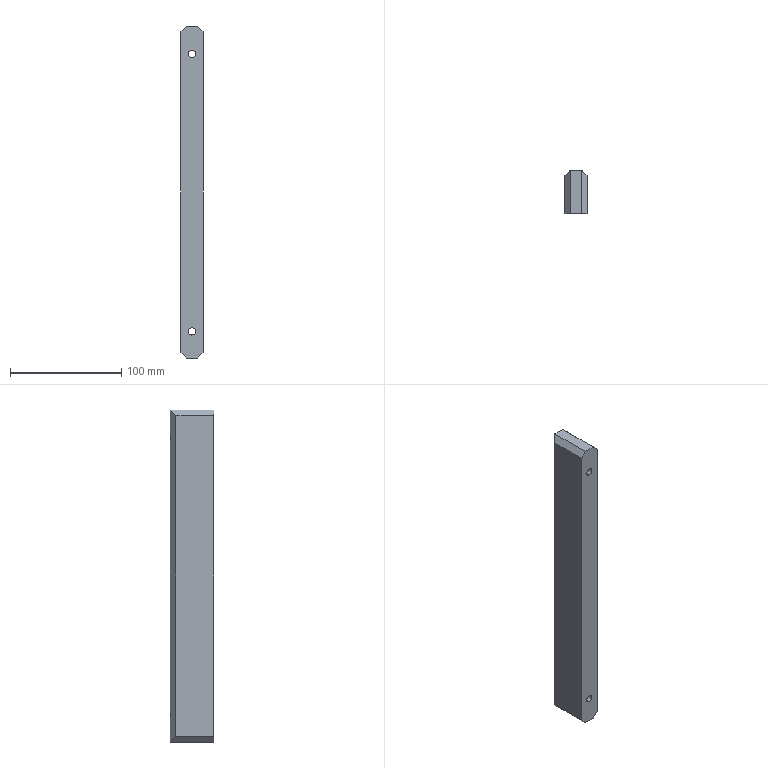Component | SolidWorks | NewDieSet-1_ReinforcingRib001-1 | 1 solid | 24 faces | box 20 x 39 x 299 mm | volume 220467 mm3 | plane 16 | cylinder 8 | commonest cylinder face diameters 11 x4 6.6 x4
STEP:
#1=COLOUR_RGB('',0.7922,0.8196,0.9333);
#2=FILL_AREA_STYLE_COLOUR('',#1);
#3=FILL_AREA_STYLE('',(#2));
#4=SURFACE_STYLE_FILL_AREA(#3);
#5=SURFACE_SIDE_STYLE('',(#4));
#6=SURFACE_STYLE_USAGE(.BOTH.,#5);
#7=PRESENTATION_STYLE_ASSIGNMENT((#6));
#8=CARTESIAN_POINT('',(0.9155,-0.03437,18.602));
#9=VERTEX_POINT('',#8);
#10=CARTESIAN_POINT('',(0.9155,-0.03437,19.035));
#11=VERTEX_POINT('',#10);
#12=CARTESIAN_POINT('',(0.9155,-0.03437,18.819));
#13=DIRECTION('',(0.,1.,0.));
#14=DIRECTION('',(0.,0.,1.));
#15=AXIS2_PLACEMENT_3D('',#12,#13,#14);
#16=CIRCLE('',#15,0.2165);
#17=EDGE_CURVE('',#9,#11,#16,.T.);
#18=ORIENTED_EDGE('',*,*,#17,.F.);
#19=CARTESIAN_POINT('',(0.9155,0.2333,18.602));
#20=VERTEX_POINT('',#19);
#21=CARTESIAN_POINT('',(0.9155,0.2333,18.602));
#22=DIRECTION('',(0.,1.,0.));
#23=VECTOR('',#22,39.37);
#24=LINE('',#21,#23);
#25=EDGE_CURVE('',#9,#20,#24,.T.);
#26=ORIENTED_EDGE('',*,*,#25,.T.);
#27=CARTESIAN_POINT('',(0.7187,0.2333,18.729));
#28=VERTEX_POINT('',#27);
#29=CARTESIAN_POINT('',(0.9155,0.2333,18.819));
#30=DIRECTION('',(0.,1.,0.));
#31=DIRECTION('',(0.,0.,1.));
#32=AXIS2_PLACEMENT_3D('',#29,#30,#31);
#33=CIRCLE('',#32,0.2165);
#34=EDGE_CURVE('',#20,#28,#33,.T.);
#35=ORIENTED_EDGE('',*,*,#34,.T.);
#36=CARTESIAN_POINT('',(0.7187,0.2333,18.909));
#37=VERTEX_POINT('',#36);
#38=CARTESIAN_POINT('',(0.7187,0.2333,18.729));
#39=CARTESIAN_POINT('',(0.692,0.2067,18.787));
#40=CARTESIAN_POINT('',(0.692,0.2067,18.851));
#41=CARTESIAN_POINT('',(0.7187,0.2333,18.909));
#42=(BOUNDED_CURVE()B_SPLINE_CURVE(3,(#38,#39,#40,#41),.UNSPECIFIED.,.F.,.T.)B_SPLINE_CURVE_WITH_KNOTS((4,4),(2.712,3.571),.UNSPECIFIED.)CURVE()GEOMETRIC_REPRESENTATION_ITEM()RATIONAL_B_SPLINE_CURVE((1.,0.9394,0.9394,1.))REPRESENTATION_ITEM(''));
#43=EDGE_CURVE('',#28,#37,#42,.T.);
#44=ORIENTED_EDGE('',*,*,#43,.T.);
#45=CARTESIAN_POINT('',(0.9155,0.2333,19.035));
#46=VERTEX_POINT('',#45);
#47=CARTESIAN_POINT('',(0.9155,0.2333,18.819));
#48=DIRECTION('',(0.,1.,0.));
#49=DIRECTION('',(0.,0.,1.));
#50=AXIS2_PLACEMENT_3D('',#47,#48,#49);
#51=CIRCLE('',#50,0.2165);
#52=EDGE_CURVE('',#37,#46,#51,.T.);
#53=ORIENTED_EDGE('',*,*,#52,.T.);
#54=CARTESIAN_POINT('',(0.9155,0.2333,19.035));
#55=DIRECTION('',(0.,1.,0.));
#56=VECTOR('',#55,39.37);
#57=LINE('',#54,#56);
#58=EDGE_CURVE('',#11,#46,#57,.T.);
#59=ORIENTED_EDGE('',*,*,#58,.F.);
#60=EDGE_LOOP('',(#18,#26,#35,#44,#53,#59));
#61=FACE_OUTER_BOUND('',#60,.T.);
#62=CARTESIAN_POINT('',(0.9155,0.2333,18.819));
#63=DIRECTION('',(0.,1.,0.));
#64=DIRECTION('',(0.,0.,1.));
#65=AXIS2_PLACEMENT_3D('',#62,#63,#64);
#66=CYLINDRICAL_SURFACE('',#65,0.2165);
#67=ADVANCED_FACE('',(#61),#66,.F.);
#68=CARTESIAN_POINT('',(0.9155,-1.302,18.689));
#69=VERTEX_POINT('',#68);
#70=CARTESIAN_POINT('',(0.9155,-1.302,18.949));
#71=VERTEX_POINT('',#70);
#72=CARTESIAN_POINT('',(0.9155,-1.302,18.819));
#73=DIRECTION('',(0.,1.,0.));
#74=DIRECTION('',(0.,0.,1.));
#75=AXIS2_PLACEMENT_3D('',#72,#73,#74);
#76=CIRCLE('',#75,0.1299);
#77=EDGE_CURVE('',#69,#71,#76,.T.);
#78=ORIENTED_EDGE('',*,*,#77,.F.);
#79=CARTESIAN_POINT('',(0.9155,-0.03437,18.689));
#80=VERTEX_POINT('',#79);
#81=CARTESIAN_POINT('',(0.9155,0.2333,18.689));
#82=DIRECTION('',(0.,1.,0.));
#83=VECTOR('',#82,39.37);
#84=LINE('',#81,#83);
#85=EDGE_CURVE('',#69,#80,#84,.T.);
#86=ORIENTED_EDGE('',*,*,#85,.T.);
#87=CARTESIAN_POINT('',(0.9155,-0.03437,18.949));
#88=VERTEX_POINT('',#87);
#89=CARTESIAN_POINT('',(0.9155,-0.03437,18.819));
#90=DIRECTION('',(0.,1.,0.));
#91=DIRECTION('',(0.,0.,1.));
#92=AXIS2_PLACEMENT_3D('',#89,#90,#91);
#93=CIRCLE('',#92,0.1299);
#94=EDGE_CURVE('',#80,#88,#93,.T.);
#95=ORIENTED_EDGE('',*,*,#94,.T.);
#96=CARTESIAN_POINT('',(0.9155,0.2333,18.949));
#97=DIRECTION('',(0.,1.,0.));
#98=VECTOR('',#97,39.37);
#99=LINE('',#96,#98);
#100=EDGE_CURVE('',#71,#88,#99,.T.);
#101=ORIENTED_EDGE('',*,*,#100,.F.);
#102=EDGE_LOOP('',(#78,#86,#95,#101));
#103=FACE_OUTER_BOUND('',#102,.T.);
#104=CARTESIAN_POINT('',(0.9155,0.2333,18.819));
#105=DIRECTION('',(0.,1.,0.));
#106=DIRECTION('',(0.,0.,1.));
#107=AXIS2_PLACEMENT_3D('',#104,#105,#106);
#108=CYLINDRICAL_SURFACE('',#107,0.1299);
#109=ADVANCED_FACE('',(#103),#108,.F.);
#110=CARTESIAN_POINT('',(0.9155,-0.03437,8.76));
#111=VERTEX_POINT('',#110);
#112=CARTESIAN_POINT('',(0.9155,-0.03437,9.193));
#113=VERTEX_POINT('',#112);
#114=CARTESIAN_POINT('',(0.9155,-0.03437,8.976));
#115=DIRECTION('',(0.,1.,0.));
#116=DIRECTION('',(0.,0.,1.));
#117=AXIS2_PLACEMENT_3D('',#114,#115,#116);
#118=CIRCLE('',#117,0.2165);
#119=EDGE_CURVE('',#111,#113,#118,.T.);
#120=ORIENTED_EDGE('',*,*,#119,.F.);
#121=CARTESIAN_POINT('',(0.9155,0.2333,8.76));
#122=VERTEX_POINT('',#121);
#123=CARTESIAN_POINT('',(0.9155,0.2333,8.76));
#124=DIRECTION('',(0.,1.,0.));
#125=VECTOR('',#124,39.37);
#126=LINE('',#123,#125);
#127=EDGE_CURVE('',#111,#122,#126,.T.);
#128=ORIENTED_EDGE('',*,*,#127,.T.);
#129=CARTESIAN_POINT('',(0.7187,0.2333,8.886));
#130=VERTEX_POINT('',#129);
#131=CARTESIAN_POINT('',(0.9155,0.2333,8.976));
#132=DIRECTION('',(0.,1.,0.));
#133=DIRECTION('',(0.,0.,1.));
#134=AXIS2_PLACEMENT_3D('',#131,#132,#133);
#135=CIRCLE('',#134,0.2165);
#136=EDGE_CURVE('',#122,#130,#135,.T.);
#137=ORIENTED_EDGE('',*,*,#136,.T.);
#138=CARTESIAN_POINT('',(0.7187,0.2333,9.067));
#139=VERTEX_POINT('',#138);
#140=CARTESIAN_POINT('',(0.7187,0.2333,8.886));
#141=CARTESIAN_POINT('',(0.692,0.2067,8.944));
#142=CARTESIAN_POINT('',(0.692,0.2067,9.008));
#143=CARTESIAN_POINT('',(0.7187,0.2333,9.067));
#144=(BOUNDED_CURVE()B_SPLINE_CURVE(3,(#140,#141,#142,#143),.UNSPECIFIED.,.F.,.T.)B_SPLINE_CURVE_WITH_KNOTS((4,4),(2.712,3.571),.UNSPECIFIED.)CURVE()GEOMETRIC_REPRESENTATION_ITEM()RATIONAL_B_SPLINE_CURVE((1.,0.9394,0.9394,1.))REPRESENTATION_ITEM(''));
#145=EDGE_CURVE('',#130,#139,#144,.T.);
#146=ORIENTED_EDGE('',*,*,#145,.T.);
#147=CARTESIAN_POINT('',(0.9155,0.2333,9.193));
#148=VERTEX_POINT('',#147);
#149=CARTESIAN_POINT('',(0.9155,0.2333,8.976));
#150=DIRECTION('',(0.,1.,0.));
#151=DIRECTION('',(0.,0.,1.));
#152=AXIS2_PLACEMENT_3D('',#149,#150,#151);
#153=CIRCLE('',#152,0.2165);
#154=EDGE_CURVE('',#139,#148,#153,.T.);
#155=ORIENTED_EDGE('',*,*,#154,.T.);
#156=CARTESIAN_POINT('',(0.9155,0.2333,9.193));
#157=DIRECTION('',(0.,1.,0.));
#158=VECTOR('',#157,39.37);
#159=LINE('',#156,#158);
#160=EDGE_CURVE('',#113,#148,#159,.T.);
#161=ORIENTED_EDGE('',*,*,#160,.F.);
#162=EDGE_LOOP('',(#120,#128,#137,#146,#155,#161));
#163=FACE_OUTER_BOUND('',#162,.T.);
#164=CARTESIAN_POINT('',(0.9155,0.2333,8.976));
#165=DIRECTION('',(0.,1.,0.));
#166=DIRECTION('',(0.,0.,1.));
#167=AXIS2_PLACEMENT_3D('',#164,#165,#166);
#168=CYLINDRICAL_SURFACE('',#167,0.2165);
#169=ADVANCED_FACE('',(#163),#168,.F.);
#170=CARTESIAN_POINT('',(0.9155,-1.302,8.846));
#171=VERTEX_POINT('',#170);
#172=CARTESIAN_POINT('',(0.9155,-1.302,9.106));
#173=VERTEX_POINT('',#172);
#174=CARTESIAN_POINT('',(0.9155,-1.302,8.976));
#175=DIRECTION('',(0.,1.,0.));
#176=DIRECTION('',(0.,0.,1.));
#177=AXIS2_PLACEMENT_3D('',#174,#175,#176);
#178=CIRCLE('',#177,0.1299);
#179=EDGE_CURVE('',#171,#173,#178,.T.);
#180=ORIENTED_EDGE('',*,*,#179,.F.);
#181=CARTESIAN_POINT('',(0.9155,-0.03437,8.846));
#182=VERTEX_POINT('',#181);
#183=CARTESIAN_POINT('',(0.9155,0.2333,8.846));
#184=DIRECTION('',(0.,1.,0.));
#185=VECTOR('',#184,39.37);
#186=LINE('',#183,#185);
#187=EDGE_CURVE('',#171,#182,#186,.T.);
#188=ORIENTED_EDGE('',*,*,#187,.T.);
#189=CARTESIAN_POINT('',(0.9155,-0.03437,9.106));
#190=VERTEX_POINT('',#189);
#191=CARTESIAN_POINT('',(0.9155,-0.03437,8.976));
#192=DIRECTION('',(0.,1.,0.));
#193=DIRECTION('',(0.,0.,1.));
#194=AXIS2_PLACEMENT_3D('',#191,#192,#193);
#195=CIRCLE('',#194,0.1299);
#196=EDGE_CURVE('',#182,#190,#195,.T.);
#197=ORIENTED_EDGE('',*,*,#196,.T.);
#198=CARTESIAN_POINT('',(0.9155,0.2333,9.106));
#199=DIRECTION('',(0.,1.,0.));
#200=VECTOR('',#199,39.37);
#201=LINE('',#198,#200);
#202=EDGE_CURVE('',#173,#190,#201,.T.);
#203=ORIENTED_EDGE('',*,*,#202,.F.);
#204=EDGE_LOOP('',(#180,#188,#197,#203));
#205=FACE_OUTER_BOUND('',#204,.T.);
#206=CARTESIAN_POINT('',(0.9155,0.2333,8.976));
#207=DIRECTION('',(0.,1.,0.));
#208=DIRECTION('',(0.,0.,1.));
#209=AXIS2_PLACEMENT_3D('',#206,#207,#208);
#210=CYLINDRICAL_SURFACE('',#209,0.1299);
#211=ADVANCED_FACE('',(#205),#210,.F.);
#212=CARTESIAN_POINT('',(1.112,0.2333,8.031));
#213=VERTEX_POINT('',#212);
#214=CARTESIAN_POINT('',(0.7187,0.2333,8.031));
#215=VERTEX_POINT('',#214);
#216=CARTESIAN_POINT('',(0.5218,0.2333,8.031));
#217=DIRECTION('',(-1.,0.,0.));
#218=VECTOR('',#217,39.37);
#219=LINE('',#216,#218);
#220=EDGE_CURVE('',#213,#215,#219,.T.);
#221=ORIENTED_EDGE('',*,*,#220,.T.);
#222=CARTESIAN_POINT('',(0.7187,0.2333,19.803));
#223=DIRECTION('',(0.,0.,1.));
#224=VECTOR('',#223,39.37);
#225=LINE('',#222,#224);
#226=EDGE_CURVE('',#215,#130,#225,.T.);
#227=ORIENTED_EDGE('',*,*,#226,.T.);
#228=ORIENTED_EDGE('',*,*,#136,.F.);
#229=CARTESIAN_POINT('',(1.112,0.2333,8.886));
#230=VERTEX_POINT('',#229);
#231=CARTESIAN_POINT('',(0.9155,0.2333,8.976));
#232=DIRECTION('',(0.,1.,0.));
#233=DIRECTION('',(0.,0.,1.));
#234=AXIS2_PLACEMENT_3D('',#231,#232,#233);
#235=CIRCLE('',#234,0.2165);
#236=EDGE_CURVE('',#230,#122,#235,.T.);
#237=ORIENTED_EDGE('',*,*,#236,.F.);
#238=CARTESIAN_POINT('',(1.112,0.2333,19.803));
#239=DIRECTION('',(0.,0.,-1.));
#240=VECTOR('',#239,39.37);
#241=LINE('',#238,#240);
#242=EDGE_CURVE('',#230,#213,#241,.T.);
#243=ORIENTED_EDGE('',*,*,#242,.T.);
#244=EDGE_LOOP('',(#221,#227,#228,#237,#243));
#245=FACE_OUTER_BOUND('',#244,.T.);
#246=CARTESIAN_POINT('',(0.5218,0.2333,19.803));
#247=DIRECTION('',(0.,-1.,0.));
#248=DIRECTION('',(0.,0.,-1.));
#249=AXIS2_PLACEMENT_3D('',#246,#247,#248);
#250=PLANE('',#249);
#251=ADVANCED_FACE('',(#245),#250,.F.);
#252=ORIENTED_EDGE('',*,*,#154,.F.);
#253=CARTESIAN_POINT('',(0.7187,0.2333,19.803));
#254=DIRECTION('',(0.,0.,1.));
#255=VECTOR('',#254,39.37);
#256=LINE('',#253,#255);
#257=EDGE_CURVE('',#139,#28,#256,.T.);
#258=ORIENTED_EDGE('',*,*,#257,.T.);
#259=ORIENTED_EDGE('',*,*,#34,.F.);
#260=CARTESIAN_POINT('',(1.112,0.2333,18.729));
#261=VERTEX_POINT('',#260);
#262=CARTESIAN_POINT('',(0.9155,0.2333,18.819));
#263=DIRECTION('',(0.,1.,0.));
#264=DIRECTION('',(0.,0.,1.));
#265=AXIS2_PLACEMENT_3D('',#262,#263,#264);
#266=CIRCLE('',#265,0.2165);
#267=EDGE_CURVE('',#261,#20,#266,.T.);
#268=ORIENTED_EDGE('',*,*,#267,.F.);
#269=CARTESIAN_POINT('',(1.112,0.2333,9.067));
#270=VERTEX_POINT('',#269);
#271=CARTESIAN_POINT('',(1.112,0.2333,19.803));
#272=DIRECTION('',(0.,0.,-1.));
#273=VECTOR('',#272,39.37);
#274=LINE('',#271,#273);
#275=EDGE_CURVE('',#261,#270,#274,.T.);
#276=ORIENTED_EDGE('',*,*,#275,.T.);
#277=CARTESIAN_POINT('',(0.9155,0.2333,8.976));
#278=DIRECTION('',(0.,1.,0.));
#279=DIRECTION('',(0.,0.,1.));
#280=AXIS2_PLACEMENT_3D('',#277,#278,#279);
#281=CIRCLE('',#280,0.2165);
#282=EDGE_CURVE('',#148,#270,#281,.T.);
#283=ORIENTED_EDGE('',*,*,#282,.F.);
#284=EDGE_LOOP('',(#252,#258,#259,#268,#276,#283));
#285=FACE_OUTER_BOUND('',#284,.T.);
#286=CARTESIAN_POINT('',(0.5218,0.2333,19.803));
#287=DIRECTION('',(0.,-1.,0.));
#288=DIRECTION('',(0.,0.,-1.));
#289=AXIS2_PLACEMENT_3D('',#286,#287,#288);
#290=PLANE('',#289);
#291=ADVANCED_FACE('',(#285),#290,.F.);
#292=CARTESIAN_POINT('',(1.309,-1.302,8.228));
#293=VERTEX_POINT('',#292);
#294=CARTESIAN_POINT('',(1.309,0.0365,8.228));
#295=VERTEX_POINT('',#294);
#296=CARTESIAN_POINT('',(1.309,0.2333,8.228));
#297=DIRECTION('',(0.,1.,0.));
#298=VECTOR('',#297,39.37);
#299=LINE('',#296,#298);
#300=EDGE_CURVE('',#293,#295,#299,.T.);
#301=ORIENTED_EDGE('',*,*,#300,.T.);
#302=CARTESIAN_POINT('',(1.309,0.0365,19.606));
#303=VERTEX_POINT('',#302);
#304=CARTESIAN_POINT('',(1.309,0.0365,19.803));
#305=DIRECTION('',(0.,0.,1.));
#306=VECTOR('',#305,39.37);
#307=LINE('',#304,#306);
#308=EDGE_CURVE('',#295,#303,#307,.T.);
#309=ORIENTED_EDGE('',*,*,#308,.T.);
#310=CARTESIAN_POINT('',(1.309,-1.302,19.606));
#311=VERTEX_POINT('',#310);
#312=CARTESIAN_POINT('',(1.309,-1.302,19.606));
#313=DIRECTION('',(0.,-1.,0.));
#314=VECTOR('',#313,39.37);
#315=LINE('',#312,#314);
#316=EDGE_CURVE('',#303,#311,#315,.T.);
#317=ORIENTED_EDGE('',*,*,#316,.T.);
#318=CARTESIAN_POINT('',(1.309,-1.302,19.803));
#319=DIRECTION('',(0.,0.,-1.));
#320=VECTOR('',#319,39.37);
#321=LINE('',#318,#320);
#322=EDGE_CURVE('',#311,#293,#321,.T.);
#323=ORIENTED_EDGE('',*,*,#322,.T.);
#324=EDGE_LOOP('',(#301,#309,#317,#323));
#325=FACE_OUTER_BOUND('',#324,.T.);
#326=CARTESIAN_POINT('',(1.309,-1.302,19.803));
#327=DIRECTION('',(-1.,0.,0.));
#328=DIRECTION('',(0.,0.,1.));
#329=AXIS2_PLACEMENT_3D('',#326,#327,#328);
#330=PLANE('',#329);
#331=ADVANCED_FACE('',(#325),#330,.F.);
#332=ORIENTED_EDGE('',*,*,#52,.F.);
#333=CARTESIAN_POINT('',(0.7187,0.2333,19.803));
#334=VERTEX_POINT('',#333);
#335=CARTESIAN_POINT('',(0.7187,0.2333,19.803));
#336=DIRECTION('',(0.,0.,1.));
#337=VECTOR('',#336,39.37);
#338=LINE('',#335,#337);
#339=EDGE_CURVE('',#37,#334,#338,.T.);
#340=ORIENTED_EDGE('',*,*,#339,.T.);
#341=CARTESIAN_POINT('',(1.112,0.2333,19.803));
#342=VERTEX_POINT('',#341);
#343=CARTESIAN_POINT('',(0.5218,0.2333,19.803));
#344=DIRECTION('',(-1.,0.,0.));
#345=VECTOR('',#344,39.37);
#346=LINE('',#343,#345);
#347=EDGE_CURVE('',#342,#334,#346,.T.);
#348=ORIENTED_EDGE('',*,*,#347,.F.);
#349=CARTESIAN_POINT('',(1.112,0.2333,18.909));
#350=VERTEX_POINT('',#349);
#351=CARTESIAN_POINT('',(1.112,0.2333,19.803));
#352=DIRECTION('',(0.,0.,-1.));
#353=VECTOR('',#352,39.37);
#354=LINE('',#351,#353);
#355=EDGE_CURVE('',#342,#350,#354,.T.);
#356=ORIENTED_EDGE('',*,*,#355,.T.);
#357=CARTESIAN_POINT('',(0.9155,0.2333,18.819));
#358=DIRECTION('',(0.,1.,0.));
#359=DIRECTION('',(0.,0.,1.));
#360=AXIS2_PLACEMENT_3D('',#357,#358,#359);
#361=CIRCLE('',#360,0.2165);
#362=EDGE_CURVE('',#46,#350,#361,.T.);
#363=ORIENTED_EDGE('',*,*,#362,.F.);
#364=EDGE_LOOP('',(#332,#340,#348,#356,#363));
#365=FACE_OUTER_BOUND('',#364,.T.);
#366=CARTESIAN_POINT('',(0.5218,0.2333,19.803));
#367=DIRECTION('',(0.,-1.,0.));
#368=DIRECTION('',(0.,0.,-1.));
#369=AXIS2_PLACEMENT_3D('',#366,#367,#368);
#370=PLANE('',#369);
#371=ADVANCED_FACE('',(#365),#370,.F.);
#372=CARTESIAN_POINT('',(0.5218,-1.302,19.606));
#373=VERTEX_POINT('',#372);
#374=CARTESIAN_POINT('',(0.5218,0.0365,19.606));
#375=VERTEX_POINT('',#374);
#376=CARTESIAN_POINT('',(0.5218,-1.302,19.606));
#377=DIRECTION('',(0.,1.,0.));
#378=VECTOR('',#377,39.37);
#379=LINE('',#376,#378);
#380=EDGE_CURVE('',#373,#375,#379,.T.);
#381=ORIENTED_EDGE('',*,*,#380,.T.);
#382=CARTESIAN_POINT('',(0.5218,0.0365,8.228));
#383=VERTEX_POINT('',#382);
#384=CARTESIAN_POINT('',(0.5218,0.0365,19.803));
#385=DIRECTION('',(0.,0.,-1.));
#386=VECTOR('',#385,39.37);
#387=LINE('',#384,#386);
#388=EDGE_CURVE('',#375,#383,#387,.T.);
#389=ORIENTED_EDGE('',*,*,#388,.T.);
#390=CARTESIAN_POINT('',(0.5218,-1.302,8.228));
#391=VERTEX_POINT('',#390);
#392=CARTESIAN_POINT('',(0.5218,-1.302,8.228));
#393=DIRECTION('',(0.,-1.,0.));
#394=VECTOR('',#393,39.37);
#395=LINE('',#392,#394);
#396=EDGE_CURVE('',#383,#391,#395,.T.);
#397=ORIENTED_EDGE('',*,*,#396,.T.);
#398=CARTESIAN_POINT('',(0.5218,-1.302,19.803));
#399=DIRECTION('',(0.,0.,-1.));
#400=VECTOR('',#399,39.37);
#401=LINE('',#398,#400);
#402=EDGE_CURVE('',#373,#391,#401,.T.);
#403=ORIENTED_EDGE('',*,*,#402,.F.);
#404=EDGE_LOOP('',(#381,#389,#397,#403));
#405=FACE_OUTER_BOUND('',#404,.T.);
#406=CARTESIAN_POINT('',(0.5218,-1.302,19.803));
#407=DIRECTION('',(1.,0.,0.));
#408=DIRECTION('',(0.,0.,-1.));
#409=AXIS2_PLACEMENT_3D('',#406,#407,#408);
#410=PLANE('',#409);
#411=ADVANCED_FACE('',(#405),#410,.F.);
#412=CARTESIAN_POINT('',(0.9155,-1.302,18.819));
#413=DIRECTION('',(0.,1.,0.));
#414=DIRECTION('',(0.,0.,1.));
#415=AXIS2_PLACEMENT_3D('',#412,#413,#414);
#416=CIRCLE('',#415,0.1299);
#417=EDGE_CURVE('',#71,#69,#416,.T.);
#418=ORIENTED_EDGE('',*,*,#417,.T.);
#419=ORIENTED_EDGE('',*,*,#77,.T.);
#420=EDGE_LOOP('',(#418,#419));
#421=FACE_BOUND('',#420,.T.);
#422=CARTESIAN_POINT('',(0.9155,-1.302,8.976));
#423=DIRECTION('',(0.,1.,0.));
#424=DIRECTION('',(0.,0.,1.));
#425=AXIS2_PLACEMENT_3D('',#422,#423,#424);
#426=CIRCLE('',#425,0.1299);
#427=EDGE_CURVE('',#173,#171,#426,.T.);
#428=ORIENTED_EDGE('',*,*,#427,.T.);
#429=ORIENTED_EDGE('',*,*,#179,.T.);
#430=EDGE_LOOP('',(#428,#429));
#431=FACE_BOUND('',#430,.T.);
#432=ORIENTED_EDGE('',*,*,#322,.F.);
#433=CARTESIAN_POINT('',(1.112,-1.302,19.803));
#434=VERTEX_POINT('',#433);
#435=CARTESIAN_POINT('',(1.112,-1.302,19.803));
#436=DIRECTION('',(-0.7071,0.,0.7071));
#437=VECTOR('',#436,39.37);
#438=LINE('',#435,#437);
#439=EDGE_CURVE('',#311,#434,#438,.T.);
#440=ORIENTED_EDGE('',*,*,#439,.T.);
#441=CARTESIAN_POINT('',(0.7187,-1.302,19.803));
#442=VERTEX_POINT('',#441);
#443=CARTESIAN_POINT('',(0.5218,-1.302,19.803));
#444=DIRECTION('',(1.,0.,0.));
#445=VECTOR('',#444,39.37);
#446=LINE('',#443,#445);
#447=EDGE_CURVE('',#442,#434,#446,.T.);
#448=ORIENTED_EDGE('',*,*,#447,.F.);
#449=CARTESIAN_POINT('',(0.7187,-1.302,19.803));
#450=DIRECTION('',(-0.7071,0.,-0.7071));
#451=VECTOR('',#450,39.37);
#452=LINE('',#449,#451);
#453=EDGE_CURVE('',#442,#373,#452,.T.);
#454=ORIENTED_EDGE('',*,*,#453,.T.);
#455=ORIENTED_EDGE('',*,*,#402,.T.);
#456=CARTESIAN_POINT('',(0.7187,-1.302,8.031));
#457=VERTEX_POINT('',#456);
#458=CARTESIAN_POINT('',(0.5218,-1.302,8.228));
#459=DIRECTION('',(0.7071,0.,-0.7071));
#460=VECTOR('',#459,39.37);
#461=LINE('',#458,#460);
#462=EDGE_CURVE('',#391,#457,#461,.T.);
#463=ORIENTED_EDGE('',*,*,#462,.T.);
#464=CARTESIAN_POINT('',(1.112,-1.302,8.031));
#465=VERTEX_POINT('',#464);
#466=CARTESIAN_POINT('',(0.5218,-1.302,8.031));
#467=DIRECTION('',(1.,0.,0.));
#468=VECTOR('',#467,39.37);
#469=LINE('',#466,#468);
#470=EDGE_CURVE('',#457,#465,#469,.T.);
#471=ORIENTED_EDGE('',*,*,#470,.T.);
#472=CARTESIAN_POINT('',(1.309,-1.302,8.228));
#473=DIRECTION('',(0.7071,0.,0.7071));
#474=VECTOR('',#473,39.37);
#475=LINE('',#472,#474);
#476=EDGE_CURVE('',#465,#293,#475,.T.);
#477=ORIENTED_EDGE('',*,*,#476,.T.);
#478=EDGE_LOOP('',(#432,#440,#448,#454,#455,#463,#471,#477));
#479=FACE_OUTER_BOUND('',#478,.T.);
#480=CARTESIAN_POINT('',(0.5218,-1.302,19.803));
#481=DIRECTION('',(0.,1.,0.));
#482=DIRECTION('',(0.,0.,1.));
#483=AXIS2_PLACEMENT_3D('',#480,#481,#482);
#484=PLANE('',#483);
#485=ADVANCED_FACE('',(#421,#431,#479),#484,.F.);
#486=ORIENTED_EDGE('',*,*,#447,.T.);
#487=CARTESIAN_POINT('',(1.112,-0.5344,19.803));
#488=DIRECTION('',(0.,1.,0.));
#489=VECTOR('',#488,39.37);
#490=LINE('',#487,#489);
#491=EDGE_CURVE('',#434,#342,#490,.T.);
#492=ORIENTED_EDGE('',*,*,#491,.T.);
#493=ORIENTED_EDGE('',*,*,#347,.T.);
#494=CARTESIAN_POINT('',(0.7187,-0.5344,19.803));
#495=DIRECTION('',(0.,-1.,0.));
#496=VECTOR('',#495,39.37);
#497=LINE('',#494,#496);
#498=EDGE_CURVE('',#334,#442,#497,.T.);
#499=ORIENTED_EDGE('',*,*,#498,.T.);
#500=EDGE_LOOP('',(#486,#492,#493,#499));
#501=FACE_OUTER_BOUND('',#500,.T.);
#502=CARTESIAN_POINT('',(0.9155,-0.5344,19.803));
#503=DIRECTION('',(0.,0.,-1.));
#504=DIRECTION('',(-1.,0.,0.));
#505=AXIS2_PLACEMENT_3D('',#502,#503,#504);
#506=PLANE('',#505);
#507=ADVANCED_FACE('',(#501),#506,.F.);
#508=ORIENTED_EDGE('',*,*,#470,.F.);
#509=CARTESIAN_POINT('',(0.7187,0.2333,8.031));
#510=DIRECTION('',(0.,1.,0.));
#511=VECTOR('',#510,39.37);
#512=LINE('',#509,#511);
#513=EDGE_CURVE('',#457,#215,#512,.T.);
#514=ORIENTED_EDGE('',*,*,#513,.T.);
#515=ORIENTED_EDGE('',*,*,#220,.F.);
#516=CARTESIAN_POINT('',(1.112,-1.302,8.031));
#517=DIRECTION('',(0.,-1.,0.));
#518=VECTOR('',#517,39.37);
#519=LINE('',#516,#518);
#520=EDGE_CURVE('',#213,#465,#519,.T.);
#521=ORIENTED_EDGE('',*,*,#520,.T.);
#522=EDGE_LOOP('',(#508,#514,#515,#521));
#523=FACE_OUTER_BOUND('',#522,.T.);
#524=CARTESIAN_POINT('',(0.9155,-0.5344,8.031));
#525=DIRECTION('',(0.,0.,-1.));
#526=DIRECTION('',(-1.,0.,0.));
#527=AXIS2_PLACEMENT_3D('',#524,#525,#526);
#528=PLANE('',#527);
#529=ADVANCED_FACE('',(#523),#528,.T.);
#530=ORIENTED_EDGE('',*,*,#316,.F.);
#531=CARTESIAN_POINT('',(1.368,-0.02256,19.547));
#532=DIRECTION('',(-0.5774,0.5774,0.5774));
#533=VECTOR('',#532,39.37);
#534=LINE('',#531,#533);
#535=EDGE_CURVE('',#303,#342,#534,.T.);
#536=ORIENTED_EDGE('',*,*,#535,.T.);
#537=ORIENTED_EDGE('',*,*,#491,.F.);
#538=ORIENTED_EDGE('',*,*,#439,.F.);
#539=EDGE_LOOP('',(#530,#536,#537,#538));
#540=FACE_OUTER_BOUND('',#539,.T.);
#541=CARTESIAN_POINT('',(1.112,-0.5344,19.803));
#542=DIRECTION('',(-0.7071,0.,-0.7071));
#543=DIRECTION('',(0.,1.,0.));
#544=AXIS2_PLACEMENT_3D('',#541,#542,#543);
#545=PLANE('',#544);
#546=ADVANCED_FACE('',(#540),#545,.F.);
#547=ORIENTED_EDGE('',*,*,#498,.F.);
#548=CARTESIAN_POINT('',(0.4627,-0.02256,19.547));
#549=DIRECTION('',(-0.5774,-0.5774,-0.5774));
#550=VECTOR('',#549,39.37);
#551=LINE('',#548,#550);
#552=EDGE_CURVE('',#334,#375,#551,.T.);
#553=ORIENTED_EDGE('',*,*,#552,.T.);
#554=ORIENTED_EDGE('',*,*,#380,.F.);
#555=ORIENTED_EDGE('',*,*,#453,.F.);
#556=EDGE_LOOP('',(#547,#553,#554,#555));
#557=FACE_OUTER_BOUND('',#556,.T.);
#558=CARTESIAN_POINT('',(0.7187,-0.5344,19.803));
#559=DIRECTION('',(0.7071,0.,-0.7071));
#560=DIRECTION('',(0.,-1.,0.));
#561=AXIS2_PLACEMENT_3D('',#558,#559,#560);
#562=PLANE('',#561);
#563=ADVANCED_FACE('',(#557),#562,.F.);
#564=ORIENTED_EDGE('',*,*,#396,.F.);
#565=CARTESIAN_POINT('',(0.07561,-0.4097,8.675));
#566=DIRECTION('',(0.5774,0.5774,-0.5774));
#567=VECTOR('',#566,39.37);
#568=LINE('',#565,#567);
#569=EDGE_CURVE('',#383,#215,#568,.T.);
#570=ORIENTED_EDGE('',*,*,#569,.T.);
#571=ORIENTED_EDGE('',*,*,#513,.F.);
#572=ORIENTED_EDGE('',*,*,#462,.F.);
#573=EDGE_LOOP('',(#564,#570,#571,#572));
#574=FACE_OUTER_BOUND('',#573,.T.);
#575=CARTESIAN_POINT('',(0.5218,-1.302,8.228));
#576=DIRECTION('',(-0.7071,0.,-0.7071));
#577=DIRECTION('',(0.,1.,0.));
#578=AXIS2_PLACEMENT_3D('',#575,#576,#577);
#579=PLANE('',#578);
#580=ADVANCED_FACE('',(#574),#579,.T.);
#581=ORIENTED_EDGE('',*,*,#520,.F.);
#582=CARTESIAN_POINT('',(1.755,-0.4097,8.675));
#583=DIRECTION('',(0.5774,-0.5774,0.5774));
#584=VECTOR('',#583,39.37);
#585=LINE('',#582,#584);
#586=EDGE_CURVE('',#213,#295,#585,.T.);
#587=ORIENTED_EDGE('',*,*,#586,.T.);
#588=ORIENTED_EDGE('',*,*,#300,.F.);
#589=ORIENTED_EDGE('',*,*,#476,.F.);
#590=EDGE_LOOP('',(#581,#587,#588,#589));
#591=FACE_OUTER_BOUND('',#590,.T.);
#592=CARTESIAN_POINT('',(1.309,-1.302,8.228));
#593=DIRECTION('',(0.7071,0.,-0.7071));
#594=DIRECTION('',(0.,-1.,0.));
#595=AXIS2_PLACEMENT_3D('',#592,#593,#594);
#596=PLANE('',#595);
#597=ADVANCED_FACE('',(#591),#596,.T.);
#598=ORIENTED_EDGE('',*,*,#187,.F.);
#599=ORIENTED_EDGE('',*,*,#427,.F.);
#600=ORIENTED_EDGE('',*,*,#202,.T.);
#601=CARTESIAN_POINT('',(0.9155,-0.03437,8.976));
#602=DIRECTION('',(0.,1.,0.));
#603=DIRECTION('',(0.,0.,1.));
#604=AXIS2_PLACEMENT_3D('',#601,#602,#603);
#605=CIRCLE('',#604,0.1299);
#606=EDGE_CURVE('',#190,#182,#605,.T.);
#607=ORIENTED_EDGE('',*,*,#606,.T.);
#608=EDGE_LOOP('',(#598,#599,#600,#607));
#609=FACE_OUTER_BOUND('',#608,.T.);
#610=CARTESIAN_POINT('',(0.9155,0.2333,8.976));
#611=DIRECTION('',(0.,1.,0.));
#612=DIRECTION('',(0.,0.,1.));
#613=AXIS2_PLACEMENT_3D('',#610,#611,#612);
#614=CYLINDRICAL_SURFACE('',#613,0.1299);
#615=ADVANCED_FACE('',(#609),#614,.F.);
#616=ORIENTED_EDGE('',*,*,#606,.F.);
#617=ORIENTED_EDGE('',*,*,#196,.F.);
#618=EDGE_LOOP('',(#616,#617));
#619=FACE_BOUND('',#618,.T.);
#620=CARTESIAN_POINT('',(0.9155,-0.03437,8.976));
#621=DIRECTION('',(0.,1.,0.));
#622=DIRECTION('',(0.,0.,1.));
#623=AXIS2_PLACEMENT_3D('',#620,#621,#622);
#624=CIRCLE('',#623,0.2165);
#625=EDGE_CURVE('',#113,#111,#624,.T.);
#626=ORIENTED_EDGE('',*,*,#625,.T.);
#627=ORIENTED_EDGE('',*,*,#119,.T.);
#628=EDGE_LOOP('',(#626,#627));
#629=FACE_OUTER_BOUND('',#628,.T.);
#630=CARTESIAN_POINT('',(1.045,-0.03437,8.976));
#631=DIRECTION('',(0.,-1.,0.));
#632=DIRECTION('',(0.,0.,-1.));
#633=AXIS2_PLACEMENT_3D('',#630,#631,#632);
#634=PLANE('',#633);
#635=ADVANCED_FACE('',(#619,#629),#634,.F.);
#636=ORIENTED_EDGE('',*,*,#127,.F.);
#637=ORIENTED_EDGE('',*,*,#625,.F.);
#638=ORIENTED_EDGE('',*,*,#160,.T.);
#639=ORIENTED_EDGE('',*,*,#282,.T.);
#640=CARTESIAN_POINT('',(1.112,0.2333,9.067));
#641=CARTESIAN_POINT('',(1.139,0.2067,9.008));
#642=CARTESIAN_POINT('',(1.139,0.2067,8.944));
#643=CARTESIAN_POINT('',(1.112,0.2333,8.886));
#644=(BOUNDED_CURVE()B_SPLINE_CURVE(3,(#640,#641,#642,#643),.UNSPECIFIED.,.F.,.T.)B_SPLINE_CURVE_WITH_KNOTS((4,4),(2.712,3.571),.UNSPECIFIED.)CURVE()GEOMETRIC_REPRESENTATION_ITEM()RATIONAL_B_SPLINE_CURVE((1.,0.9394,0.9394,1.))REPRESENTATION_ITEM(''));
#645=EDGE_CURVE('',#270,#230,#644,.T.);
#646=ORIENTED_EDGE('',*,*,#645,.T.);
#647=ORIENTED_EDGE('',*,*,#236,.T.);
#648=EDGE_LOOP('',(#636,#637,#638,#639,#646,#647));
#649=FACE_OUTER_BOUND('',#648,.T.);
#650=CARTESIAN_POINT('',(0.9155,0.2333,8.976));
#651=DIRECTION('',(0.,1.,0.));
#652=DIRECTION('',(0.,0.,1.));
#653=AXIS2_PLACEMENT_3D('',#650,#651,#652);
#654=CYLINDRICAL_SURFACE('',#653,0.2165);
#655=ADVANCED_FACE('',(#649),#654,.F.);
#656=ORIENTED_EDGE('',*,*,#85,.F.);
#657=ORIENTED_EDGE('',*,*,#417,.F.);
#658=ORIENTED_EDGE('',*,*,#100,.T.);
#659=CARTESIAN_POINT('',(0.9155,-0.03437,18.819));
#660=DIRECTION('',(0.,1.,0.));
#661=DIRECTION('',(0.,0.,1.));
#662=AXIS2_PLACEMENT_3D('',#659,#660,#661);
#663=CIRCLE('',#662,0.1299);
#664=EDGE_CURVE('',#88,#80,#663,.T.);
#665=ORIENTED_EDGE('',*,*,#664,.T.);
#666=EDGE_LOOP('',(#656,#657,#658,#665));
#667=FACE_OUTER_BOUND('',#666,.T.);
#668=CARTESIAN_POINT('',(0.9155,0.2333,18.819));
#669=DIRECTION('',(0.,1.,0.));
#670=DIRECTION('',(0.,0.,1.));
#671=AXIS2_PLACEMENT_3D('',#668,#669,#670);
#672=CYLINDRICAL_SURFACE('',#671,0.1299);
#673=ADVANCED_FACE('',(#667),#672,.F.);
#674=ORIENTED_EDGE('',*,*,#664,.F.);
#675=ORIENTED_EDGE('',*,*,#94,.F.);
#676=EDGE_LOOP('',(#674,#675));
#677=FACE_BOUND('',#676,.T.);
#678=CARTESIAN_POINT('',(0.9155,-0.03437,18.819));
#679=DIRECTION('',(0.,1.,0.));
#680=DIRECTION('',(0.,0.,1.));
#681=AXIS2_PLACEMENT_3D('',#678,#679,#680);
#682=CIRCLE('',#681,0.2165);
#683=EDGE_CURVE('',#11,#9,#682,.T.);
#684=ORIENTED_EDGE('',*,*,#683,.T.);
#685=ORIENTED_EDGE('',*,*,#17,.T.);
#686=EDGE_LOOP('',(#684,#685));
#687=FACE_OUTER_BOUND('',#686,.T.);
#688=CARTESIAN_POINT('',(1.045,-0.03437,18.819));
#689=DIRECTION('',(0.,-1.,0.));
#690=DIRECTION('',(0.,0.,-1.));
#691=AXIS2_PLACEMENT_3D('',#688,#689,#690);
#692=PLANE('',#691);
#693=ADVANCED_FACE('',(#677,#687),#692,.F.);
#694=ORIENTED_EDGE('',*,*,#25,.F.);
#695=ORIENTED_EDGE('',*,*,#683,.F.);
#696=ORIENTED_EDGE('',*,*,#58,.T.);
#697=ORIENTED_EDGE('',*,*,#362,.T.);
#698=CARTESIAN_POINT('',(1.112,0.2333,18.909));
#699=CARTESIAN_POINT('',(1.139,0.2067,18.851));
#700=CARTESIAN_POINT('',(1.139,0.2067,18.787));
#701=CARTESIAN_POINT('',(1.112,0.2333,18.729));
#702=(BOUNDED_CURVE()B_SPLINE_CURVE(3,(#698,#699,#700,#701),.UNSPECIFIED.,.F.,.T.)B_SPLINE_CURVE_WITH_KNOTS((4,4),(2.712,3.571),.UNSPECIFIED.)CURVE()GEOMETRIC_REPRESENTATION_ITEM()RATIONAL_B_SPLINE_CURVE((1.,0.9394,0.9394,1.))REPRESENTATION_ITEM(''));
#703=EDGE_CURVE('',#350,#261,#702,.T.);
#704=ORIENTED_EDGE('',*,*,#703,.T.);
#705=ORIENTED_EDGE('',*,*,#267,.T.);
#706=EDGE_LOOP('',(#694,#695,#696,#697,#704,#705));
#707=FACE_OUTER_BOUND('',#706,.T.);
#708=CARTESIAN_POINT('',(0.9155,0.2333,18.819));
#709=DIRECTION('',(0.,1.,0.));
#710=DIRECTION('',(0.,0.,1.));
#711=AXIS2_PLACEMENT_3D('',#708,#709,#710);
#712=CYLINDRICAL_SURFACE('',#711,0.2165);
#713=ADVANCED_FACE('',(#707),#712,.F.);
#714=ORIENTED_EDGE('',*,*,#145,.F.);
#715=ORIENTED_EDGE('',*,*,#226,.F.);
#716=ORIENTED_EDGE('',*,*,#569,.F.);
#717=ORIENTED_EDGE('',*,*,#388,.F.);
#718=ORIENTED_EDGE('',*,*,#552,.F.);
#719=ORIENTED_EDGE('',*,*,#339,.F.);
#720=ORIENTED_EDGE('',*,*,#43,.F.);
#721=ORIENTED_EDGE('',*,*,#257,.F.);
#722=EDGE_LOOP('',(#714,#715,#716,#717,#718,#719,#720,#721));
#723=FACE_OUTER_BOUND('',#722,.T.);
#724=CARTESIAN_POINT('',(0.5218,0.0365,19.803));
#725=DIRECTION('',(0.7071,-0.7071,0.));
#726=DIRECTION('',(0.,0.,-1.));
#727=AXIS2_PLACEMENT_3D('',#724,#725,#726);
#728=PLANE('',#727);
#729=ADVANCED_FACE('',(#723),#728,.F.);
#730=ORIENTED_EDGE('',*,*,#535,.F.);
#731=ORIENTED_EDGE('',*,*,#308,.F.);
#732=ORIENTED_EDGE('',*,*,#586,.F.);
#733=ORIENTED_EDGE('',*,*,#242,.F.);
#734=ORIENTED_EDGE('',*,*,#645,.F.);
#735=ORIENTED_EDGE('',*,*,#275,.F.);
#736=ORIENTED_EDGE('',*,*,#703,.F.);
#737=ORIENTED_EDGE('',*,*,#355,.F.);
#738=EDGE_LOOP('',(#730,#731,#732,#733,#734,#735,#736,#737));
#739=FACE_OUTER_BOUND('',#738,.T.);
#740=CARTESIAN_POINT('',(1.112,0.2333,19.803));
#741=DIRECTION('',(-0.7071,-0.7071,0.));
#742=DIRECTION('',(0.,0.,-1.));
#743=AXIS2_PLACEMENT_3D('',#740,#741,#742);
#744=PLANE('',#743);
#745=ADVANCED_FACE('',(#739),#744,.F.);
#746=CLOSED_SHELL('',(#67,#109,#169,#211,#251,#291,#331,#371,#411,#485,#507,#529,#546,#563,#580,#597,#615,#635,#655,#673,#693,#713,#729,#745));
#747=MANIFOLD_SOLID_BREP('',#746);
#748=STYLED_ITEM('',(#7),#747);
#749=(LENGTH_UNIT()NAMED_UNIT(*)SI_UNIT($,.METRE.));
#750=LENGTH_MEASURE_WITH_UNIT(LENGTH_MEASURE(0.0254),#749);
#751=DIMENSIONAL_EXPONENTS(1.,0.,0.,0.,0.,0.,0.);
#752=(CONVERSION_BASED_UNIT('',#750)LENGTH_UNIT()NAMED_UNIT(#751));
#753=UNCERTAINTY_MEASURE_WITH_UNIT(LENGTH_MEASURE(0.00001),#752,'','');
#754=(NAMED_UNIT(*)PLANE_ANGLE_UNIT()SI_UNIT($,.RADIAN.));
#755=(NAMED_UNIT(*)SI_UNIT($,.STERADIAN.)SOLID_ANGLE_UNIT());
#756=(GEOMETRIC_REPRESENTATION_CONTEXT(3)GLOBAL_UNCERTAINTY_ASSIGNED_CONTEXT((#753))GLOBAL_UNIT_ASSIGNED_CONTEXT((#752,#754,#755))REPRESENTATION_CONTEXT('',''));
#757=MECHANICAL_DESIGN_GEOMETRIC_PRESENTATION_REPRESENTATION('',(#748),#756);
#758=PRESENTATION_LAYER_ASSIGNMENT('','',(#748));
#759=CARTESIAN_POINT('',(0.,0.,0.));
#760=DIRECTION('',(0.,0.,1.));
#761=DIRECTION('',(1.,0.,0.));
#762=AXIS2_PLACEMENT_3D('',#759,#760,#761);
#763=(LENGTH_UNIT()NAMED_UNIT(*)SI_UNIT($,.METRE.));
#764=LENGTH_MEASURE_WITH_UNIT(LENGTH_MEASURE(0.0254),#763);
#765=DIMENSIONAL_EXPONENTS(1.,0.,0.,0.,0.,0.,0.);
#766=(CONVERSION_BASED_UNIT('',#764)LENGTH_UNIT()NAMED_UNIT(#765));
#767=UNCERTAINTY_MEASURE_WITH_UNIT(LENGTH_MEASURE(0.00001),#766,'','');
#768=(NAMED_UNIT(*)PLANE_ANGLE_UNIT()SI_UNIT($,.RADIAN.));
#769=(NAMED_UNIT(*)SI_UNIT($,.STERADIAN.)SOLID_ANGLE_UNIT());
#770=(GEOMETRIC_REPRESENTATION_CONTEXT(3)GLOBAL_UNCERTAINTY_ASSIGNED_CONTEXT((#767))GLOBAL_UNIT_ASSIGNED_CONTEXT((#766,#768,#769))REPRESENTATION_CONTEXT('',''));
#771=ADVANCED_BREP_SHAPE_REPRESENTATION('',(#747,#762),#770);